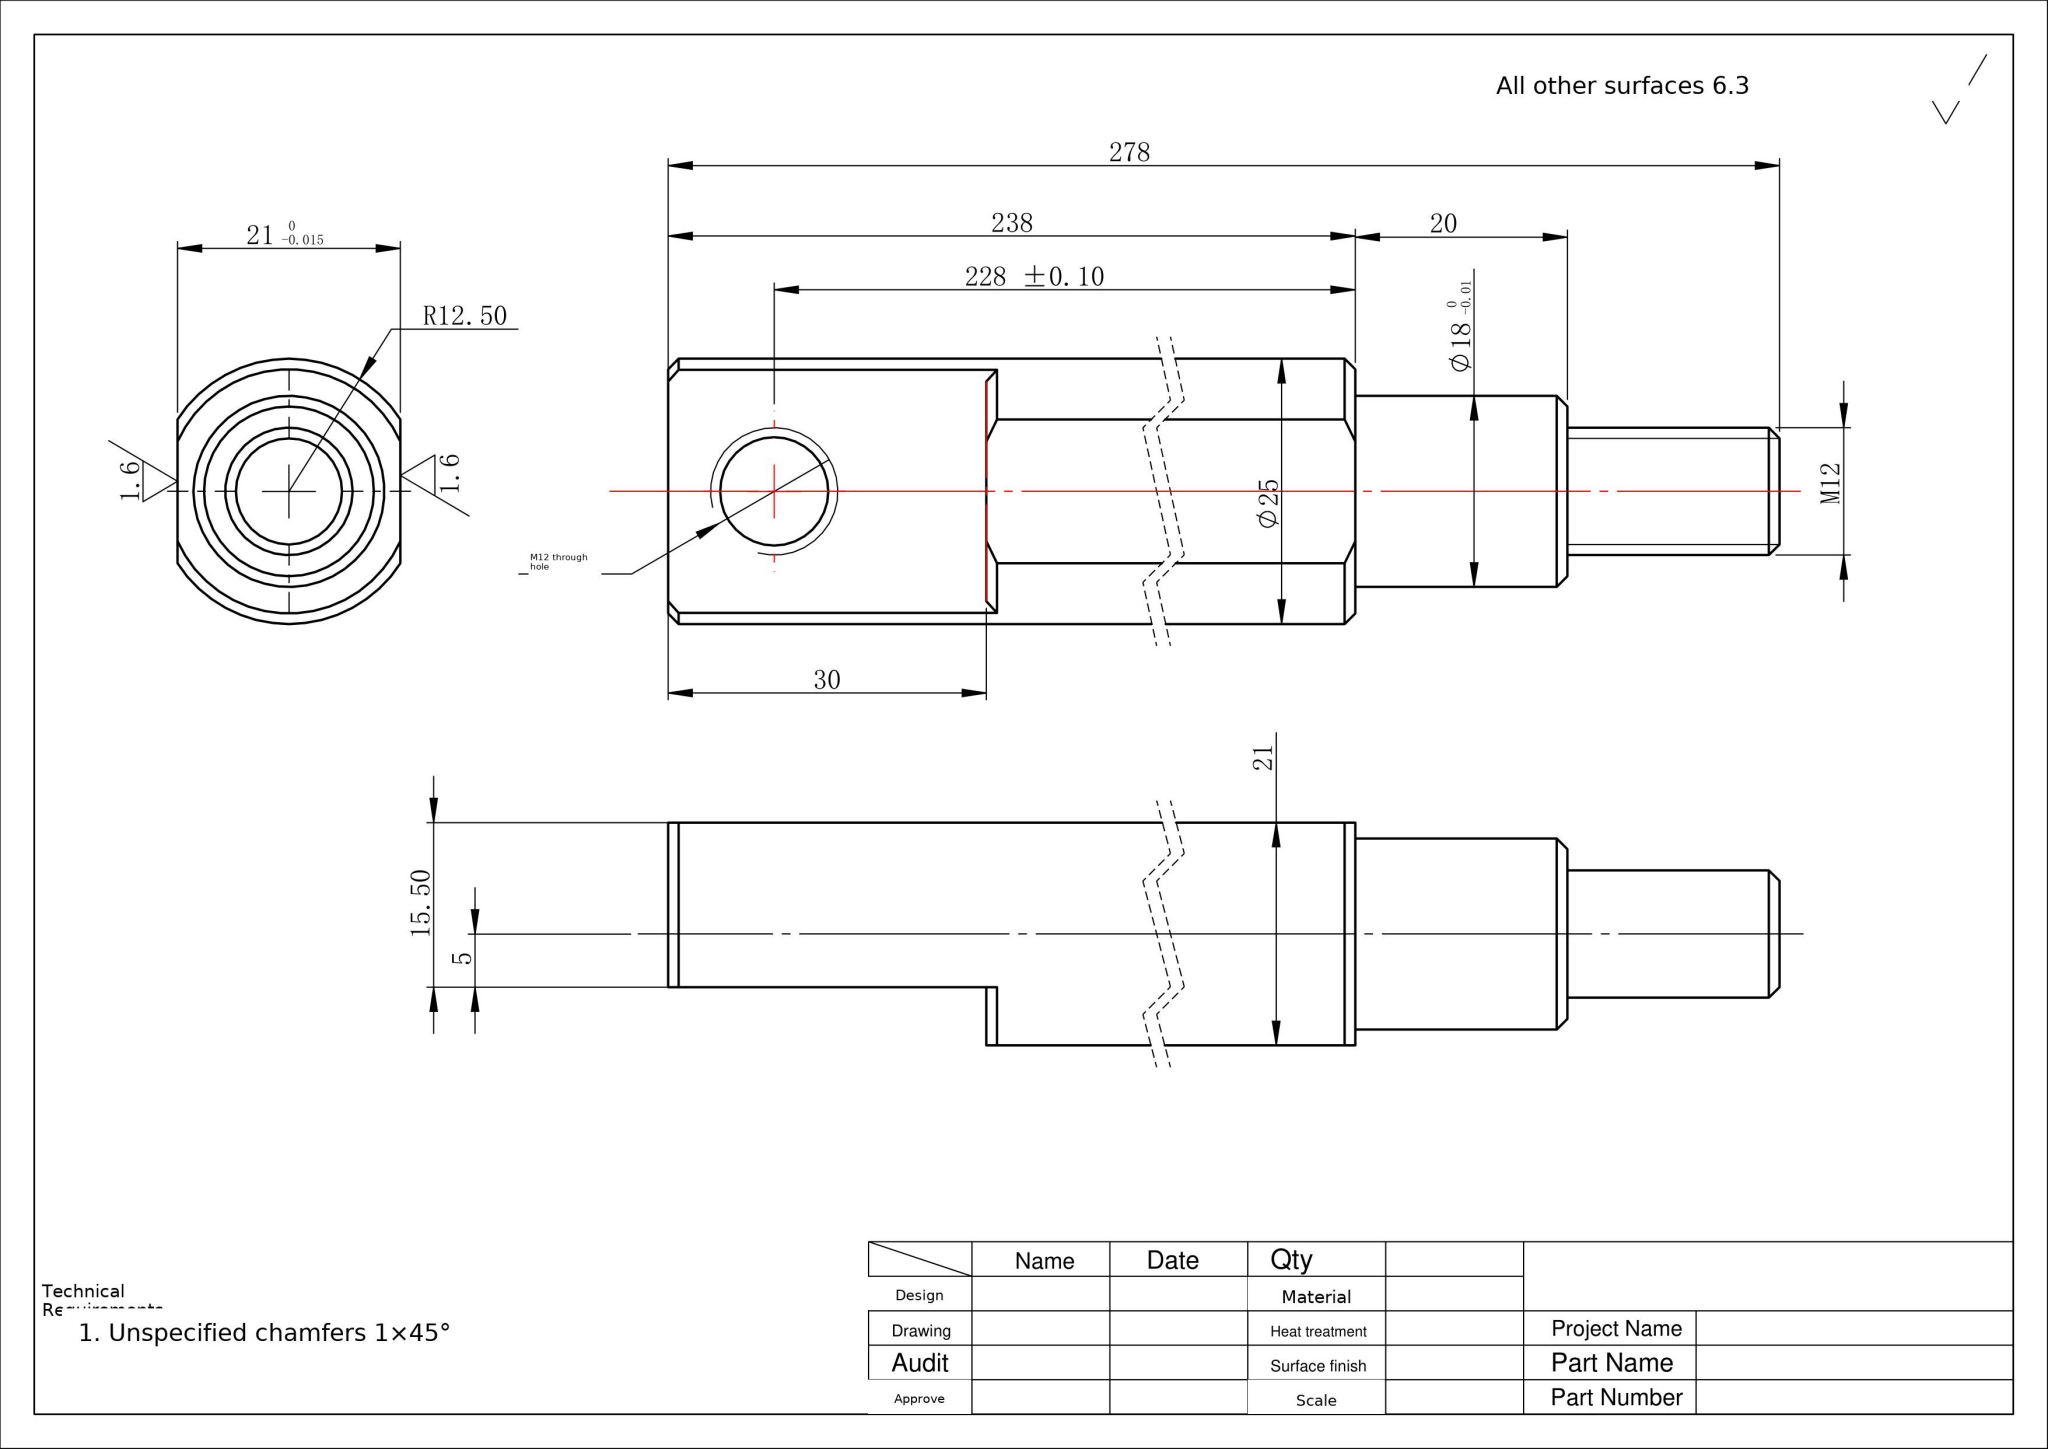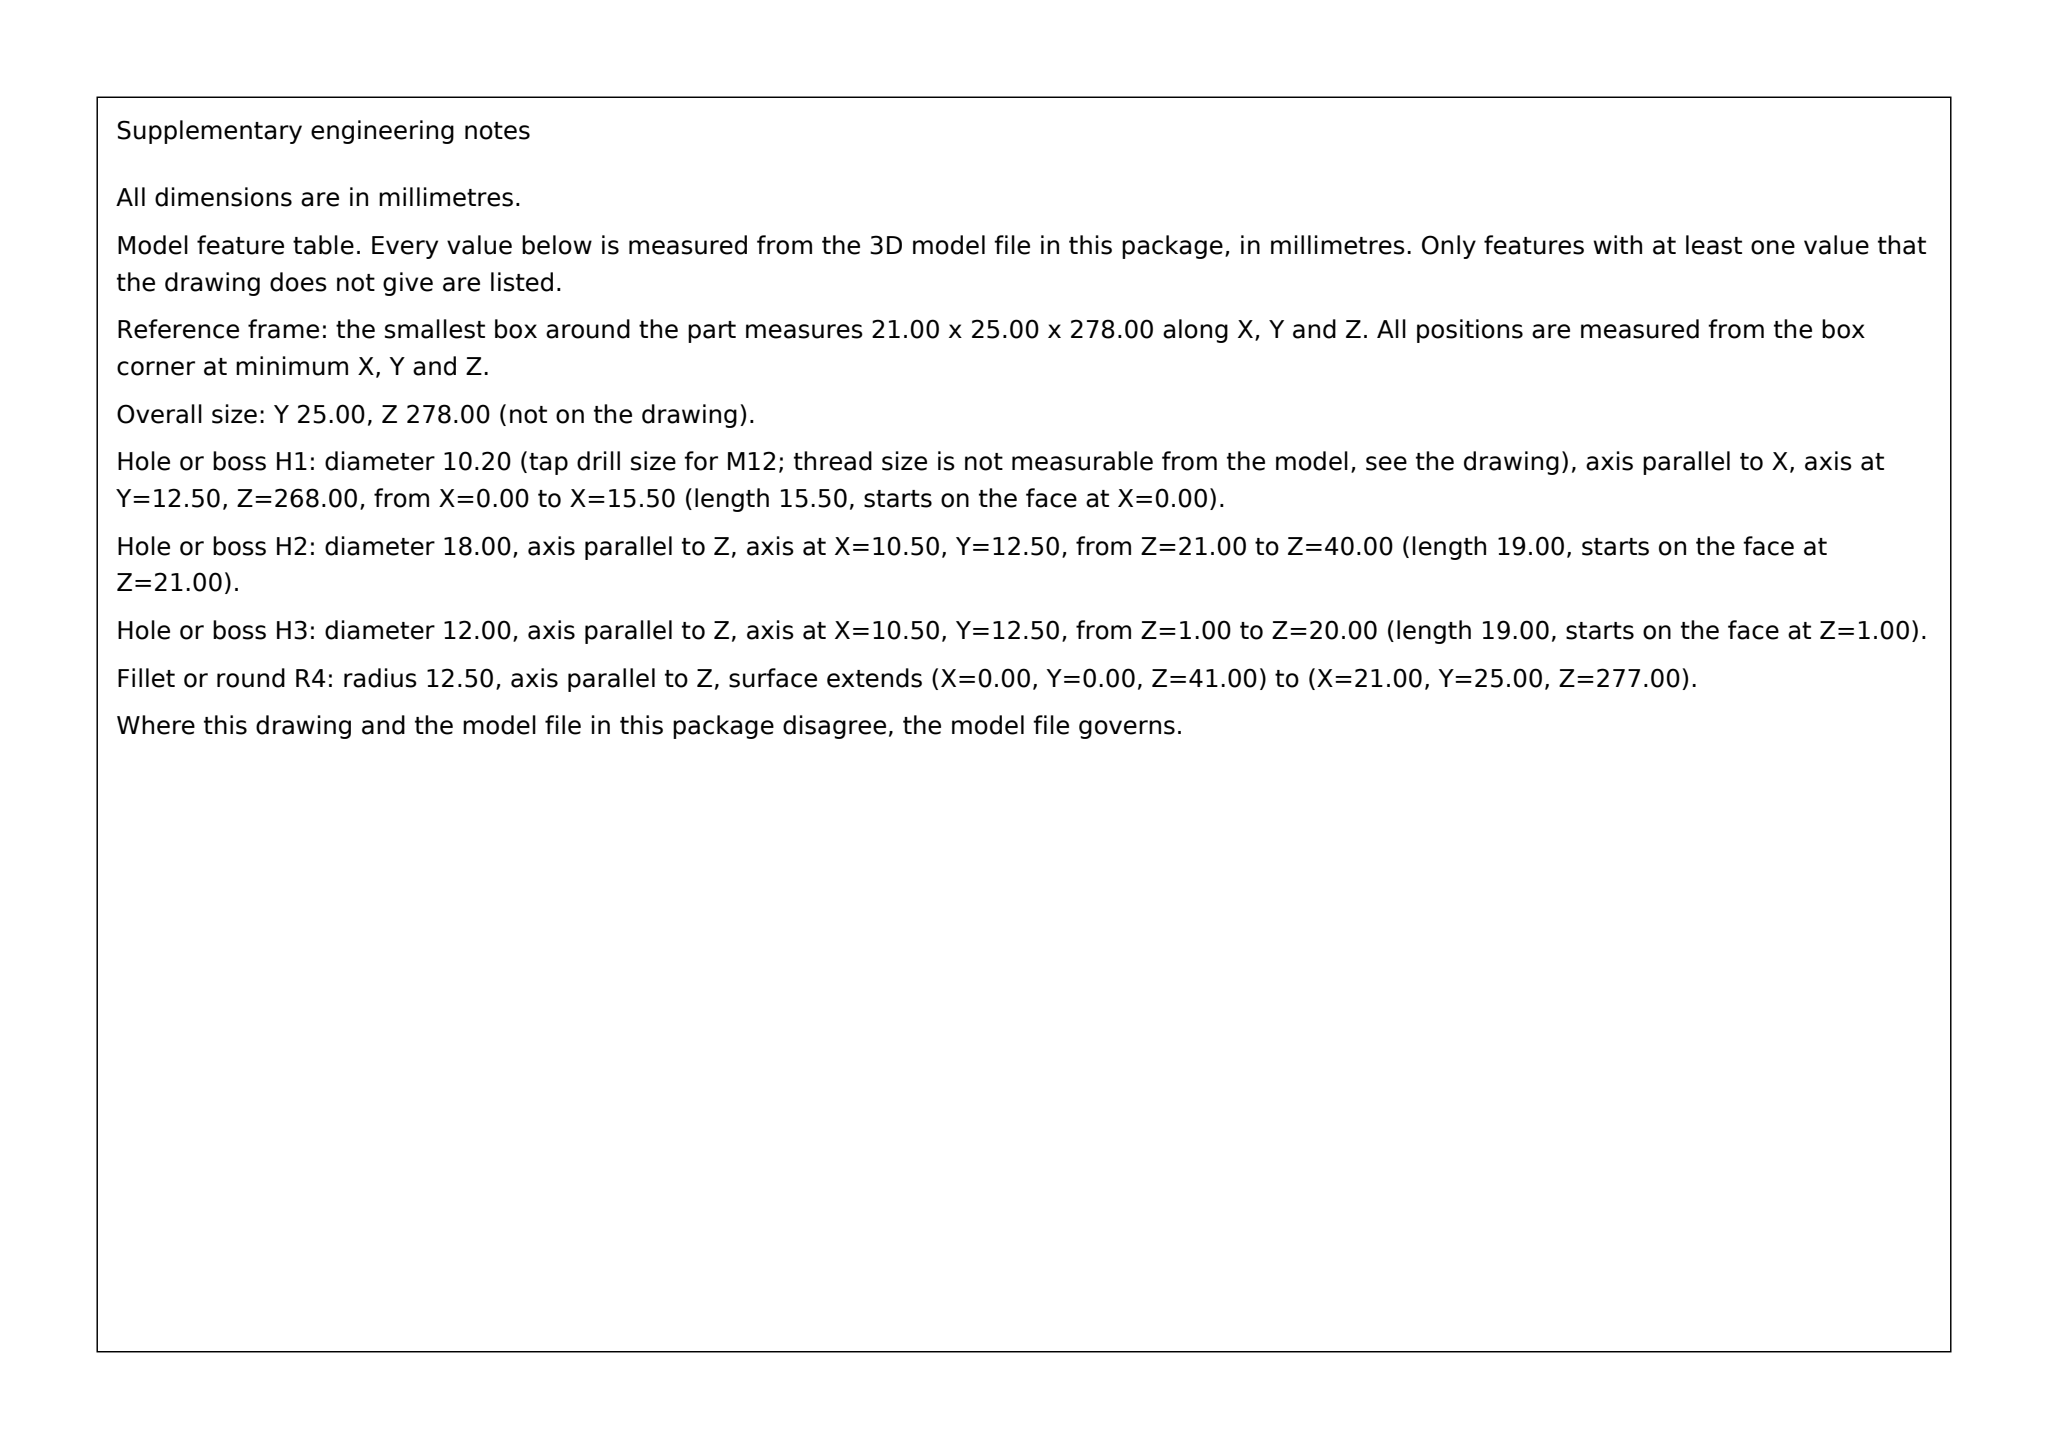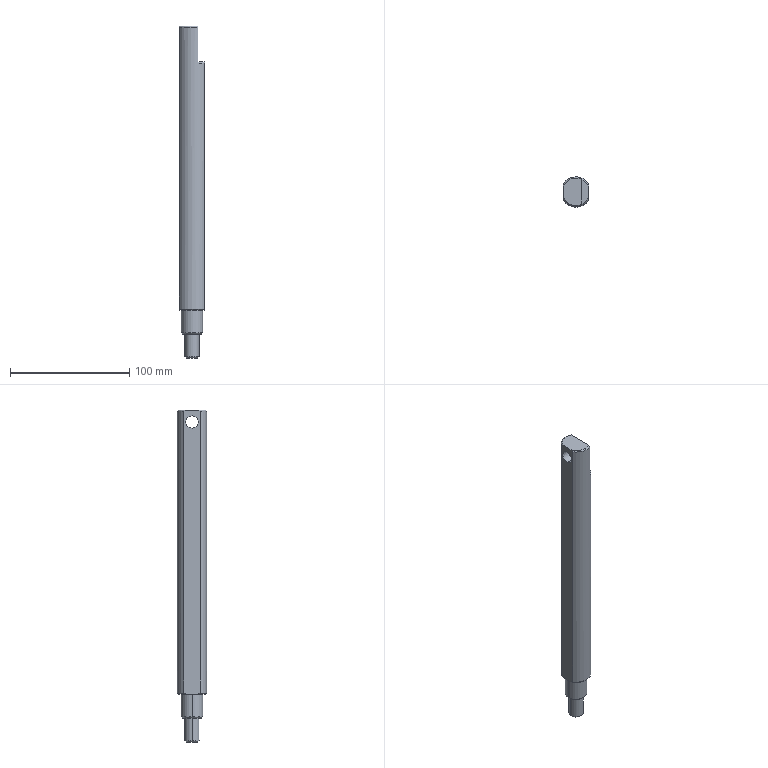Part | SolidWorks | 1 solid | 26 faces | box 21 x 25 x 278 mm | volume 110896 mm3 | cone 10 | cylinder 8 | plane 8 | commonest cylinder face diameters 12 x2 10.2 x2 18 x2 25 x2
build123d program:
from build123d import *

# Parameters (mm, degrees)
SKETCH1_R          = 9
EXTRUDE1_DEPTH     = 20
SKETCH2_R          = 12.5
EXTRUDE2_DEPTH     = 238
SKETCH6_W          = 409.623
SKETCH6_H          = 160.738
CUT_EXTRUDE2_DEPTH = 2
SKETCH7_W          = 385.784
SKETCH7_H          = 115.789
CUT_EXTRUDE3_DEPTH = 2
SKETCH8_W          = 72.586
SKETCH8_H          = 57.889
CUT_EXTRUDE4_DEPTH = 5.5
M12_TAPPED_HOLE2_D = 10.2
SKETCH11_R         = 6
EXTRUDE4_DEPTH     = 20
CHAMFER1_SIZE      = 1


with BuildPart() as part:
    # Sketch1 → Extrude1 (new body)
    with BuildSketch(Plane.XY):
        Circle(SKETCH1_R)
    extrude(amount=EXTRUDE1_DEPTH)

    # Sketch2 → Extrude2 (add)
    with BuildSketch(Plane.XY.offset(20)):
        Circle(SKETCH2_R)
    extrude(amount=EXTRUDE2_DEPTH)

    # Sketch6 → Cut-Extrude2 (cut)
    with BuildSketch(Plane(origin=(12.5, 0, 0), x_dir=(0, 0, -1), z_dir=(1, 0, 0))):
        with Locations((-133.648, -11.686)):
            Rectangle(SKETCH6_W, SKETCH6_H)
    extrude(amount=-CUT_EXTRUDE2_DEPTH, mode=Mode.SUBTRACT)

    # Sketch7 → Cut-Extrude3 (cut)
    with BuildSketch(Plane(origin=(-12.5, 0, 0), x_dir=(0, 0, -1), z_dir=(1, 0, 0))):
        with Locations((-137.977, 12.933)):
            Rectangle(SKETCH7_W, SKETCH7_H)
    extrude(amount=CUT_EXTRUDE3_DEPTH, mode=Mode.SUBTRACT)

    # Sketch8 → Cut-Extrude4 (cut)
    with BuildSketch(Plane(origin=(10.5, 0, 0), x_dir=(0, 0, -1), z_dir=(1, 0, 0))):
        with Locations((-264.293, -0.1573)):
            Rectangle(SKETCH8_W, SKETCH8_H)
    extrude(amount=-CUT_EXTRUDE4_DEPTH, mode=Mode.SUBTRACT)

    # M12 Tapped Hole2 (through all)
    with Locations(Plane(origin=(5, 0, 248), x_dir=(0, 0, 1), z_dir=(1, 0, 0))):
        with Locations((0, 0)):
            Hole(M12_TAPPED_HOLE2_D / 2)

    # Sketch11 → Extrude4 (add)
    with BuildSketch(Plane(origin=(0, 0, 0), x_dir=(-1, 0, 0), z_dir=(0, 0, -1))):
        with Locations(Location((0, 0, 0), (0, 0, 180))):
            Circle(SKETCH11_R)
    extrude(amount=EXTRUDE4_DEPTH)

    # Chamfer1
    chamfer1_edges = [part.edges().sort_by_distance(p)[0] for p in [
        (0, 12.5, 20),
        (-9, 0, 0),
        (-3.609, -11.968, 258),
        (0, -12.5, 20),
        (-3.609, 11.968, 258),
        (8.095, 9.525, 228),
        (8.095, -9.525, 228),
        (-6, 0, -20),
    ]]
    chamfer(chamfer1_edges, length=CHAMFER1_SIZE)


solid = part.part
STEP:
#1=CARTESIAN_POINT('',(-8.,0.,0.));
#2=VERTEX_POINT('',#1);
#3=CARTESIAN_POINT('',(8.,0.,0.));
#4=VERTEX_POINT('',#3);
#5=CARTESIAN_POINT('',(0.,0.,0.));
#6=DIRECTION('',(0.,0.,-1.));
#7=DIRECTION('',(1.,0.,0.));
#8=AXIS2_PLACEMENT_3D('',#5,#6,#7);
#9=CIRCLE('',#8,8.);
#10=EDGE_CURVE('',#2,#4,#9,.T.);
#11=ORIENTED_EDGE('',*,*,#10,.F.);
#12=CARTESIAN_POINT('',(-9.,0.,1.));
#13=VERTEX_POINT('',#12);
#14=CARTESIAN_POINT('',(-9.,0.,1.));
#15=DIRECTION('',(-0.7071,0.,0.7071));
#16=VECTOR('',#15,1000.);
#17=LINE('',#14,#16);
#18=EDGE_CURVE('',#2,#13,#17,.T.);
#19=ORIENTED_EDGE('',*,*,#18,.T.);
#20=CARTESIAN_POINT('',(9.,0.,1.));
#21=VERTEX_POINT('',#20);
#22=CARTESIAN_POINT('',(0.,0.,1.));
#23=DIRECTION('',(0.,0.,1.));
#24=DIRECTION('',(1.,0.,0.));
#25=AXIS2_PLACEMENT_3D('',#22,#23,#24);
#26=CIRCLE('',#25,9.);
#27=EDGE_CURVE('',#21,#13,#26,.T.);
#28=ORIENTED_EDGE('',*,*,#27,.F.);
#29=CARTESIAN_POINT('',(9.,0.,1.));
#30=DIRECTION('',(0.7071,0.,0.7071));
#31=VECTOR('',#30,1000.);
#32=LINE('',#29,#31);
#33=EDGE_CURVE('',#4,#21,#32,.T.);
#34=ORIENTED_EDGE('',*,*,#33,.F.);
#35=EDGE_LOOP('',(#11,#19,#28,#34));
#36=FACE_OUTER_BOUND('',#35,.T.);
#37=CARTESIAN_POINT('',(0.,0.,1.));
#38=DIRECTION('',(0.,0.,1.));
#39=DIRECTION('',(1.,0.,0.));
#40=AXIS2_PLACEMENT_3D('',#37,#38,#39);
#41=CONICAL_SURFACE('',#40,9.,0.7854);
#42=ADVANCED_FACE('',(#36),#41,.T.);
#43=CARTESIAN_POINT('',(-5.,0.,-20.));
#44=VERTEX_POINT('',#43);
#45=CARTESIAN_POINT('',(5.,0.,-20.));
#46=VERTEX_POINT('',#45);
#47=CARTESIAN_POINT('',(0.,0.,-20.));
#48=DIRECTION('',(0.,0.,-1.));
#49=DIRECTION('',(-1.,0.,0.));
#50=AXIS2_PLACEMENT_3D('',#47,#48,#49);
#51=CIRCLE('',#50,5.);
#52=EDGE_CURVE('',#44,#46,#51,.T.);
#53=ORIENTED_EDGE('',*,*,#52,.F.);
#54=CARTESIAN_POINT('',(-6.,0.,-19.));
#55=VERTEX_POINT('',#54);
#56=CARTESIAN_POINT('',(-5.,0.,-20.));
#57=DIRECTION('',(-0.7071,0.,0.7071));
#58=VECTOR('',#57,1000.);
#59=LINE('',#56,#58);
#60=EDGE_CURVE('',#44,#55,#59,.T.);
#61=ORIENTED_EDGE('',*,*,#60,.T.);
#62=CARTESIAN_POINT('',(6.,0.,-19.));
#63=VERTEX_POINT('',#62);
#64=CARTESIAN_POINT('',(0.,0.,-19.));
#65=DIRECTION('',(0.,0.,1.));
#66=DIRECTION('',(-1.,0.,0.));
#67=AXIS2_PLACEMENT_3D('',#64,#65,#66);
#68=CIRCLE('',#67,6.);
#69=EDGE_CURVE('',#63,#55,#68,.T.);
#70=ORIENTED_EDGE('',*,*,#69,.F.);
#71=CARTESIAN_POINT('',(5.,0.,-20.));
#72=DIRECTION('',(0.7071,0.,0.7071));
#73=VECTOR('',#72,1000.);
#74=LINE('',#71,#73);
#75=EDGE_CURVE('',#46,#63,#74,.T.);
#76=ORIENTED_EDGE('',*,*,#75,.F.);
#77=EDGE_LOOP('',(#53,#61,#70,#76));
#78=FACE_OUTER_BOUND('',#77,.T.);
#79=CARTESIAN_POINT('',(0.,0.,-20.));
#80=DIRECTION('',(0.,0.,1.));
#81=DIRECTION('',(1.,0.,0.));
#82=AXIS2_PLACEMENT_3D('',#79,#80,#81);
#83=CONICAL_SURFACE('',#82,5.,0.7854);
#84=ADVANCED_FACE('',(#78),#83,.T.);
#85=ORIENTED_EDGE('',*,*,#69,.T.);
#86=CARTESIAN_POINT('',(-6.,0.,0.));
#87=VERTEX_POINT('',#86);
#88=CARTESIAN_POINT('',(-6.,0.,-20.));
#89=DIRECTION('',(0.,0.,1.));
#90=VECTOR('',#89,1000.);
#91=LINE('',#88,#90);
#92=EDGE_CURVE('',#55,#87,#91,.T.);
#93=ORIENTED_EDGE('',*,*,#92,.T.);
#94=CARTESIAN_POINT('',(6.,0.,0.));
#95=VERTEX_POINT('',#94);
#96=CARTESIAN_POINT('',(0.,0.,0.));
#97=DIRECTION('',(0.,0.,-1.));
#98=DIRECTION('',(1.,0.,0.));
#99=AXIS2_PLACEMENT_3D('',#96,#97,#98);
#100=CIRCLE('',#99,6.);
#101=EDGE_CURVE('',#87,#95,#100,.T.);
#102=ORIENTED_EDGE('',*,*,#101,.T.);
#103=CARTESIAN_POINT('',(6.,0.,-20.));
#104=DIRECTION('',(0.,0.,1.));
#105=VECTOR('',#104,1000.);
#106=LINE('',#103,#105);
#107=EDGE_CURVE('',#63,#95,#106,.T.);
#108=ORIENTED_EDGE('',*,*,#107,.F.);
#109=EDGE_LOOP('',(#85,#93,#102,#108));
#110=FACE_OUTER_BOUND('',#109,.T.);
#111=CARTESIAN_POINT('',(0.,0.,-20.));
#112=DIRECTION('',(0.,0.,1.));
#113=DIRECTION('',(1.,0.,0.));
#114=AXIS2_PLACEMENT_3D('',#111,#112,#113);
#115=CYLINDRICAL_SURFACE('',#114,6.);
#116=ADVANCED_FACE('',(#110),#115,.T.);
#117=CARTESIAN_POINT('',(-10.5,0.,253.1));
#118=VERTEX_POINT('',#117);
#119=CARTESIAN_POINT('',(-10.5,0.,242.9));
#120=VERTEX_POINT('',#119);
#121=CARTESIAN_POINT('',(-10.5,0.,248.));
#122=DIRECTION('',(1.,0.,0.));
#123=DIRECTION('',(0.,0.,-1.));
#124=AXIS2_PLACEMENT_3D('',#121,#122,#123);
#125=CIRCLE('',#124,5.1);
#126=EDGE_CURVE('',#118,#120,#125,.T.);
#127=ORIENTED_EDGE('',*,*,#126,.F.);
#128=CARTESIAN_POINT('',(5.,0.,253.1));
#129=VERTEX_POINT('',#128);
#130=CARTESIAN_POINT('',(5.,0.,253.1));
#131=DIRECTION('',(1.,0.,0.));
#132=VECTOR('',#131,1000.);
#133=LINE('',#130,#132);
#134=EDGE_CURVE('',#118,#129,#133,.T.);
#135=ORIENTED_EDGE('',*,*,#134,.T.);
#136=CARTESIAN_POINT('',(5.,0.,242.9));
#137=VERTEX_POINT('',#136);
#138=CARTESIAN_POINT('',(5.,0.,248.));
#139=DIRECTION('',(1.,0.,0.));
#140=DIRECTION('',(0.,0.,-1.));
#141=AXIS2_PLACEMENT_3D('',#138,#139,#140);
#142=CIRCLE('',#141,5.1);
#143=EDGE_CURVE('',#129,#137,#142,.T.);
#144=ORIENTED_EDGE('',*,*,#143,.T.);
#145=CARTESIAN_POINT('',(5.,0.,242.9));
#146=DIRECTION('',(1.,0.,0.));
#147=VECTOR('',#146,1000.);
#148=LINE('',#145,#147);
#149=EDGE_CURVE('',#120,#137,#148,.T.);
#150=ORIENTED_EDGE('',*,*,#149,.F.);
#151=EDGE_LOOP('',(#127,#135,#144,#150));
#152=FACE_OUTER_BOUND('',#151,.T.);
#153=CARTESIAN_POINT('',(5.,0.,248.));
#154=DIRECTION('',(1.,0.,0.));
#155=DIRECTION('',(0.,0.,-1.));
#156=AXIS2_PLACEMENT_3D('',#153,#154,#155);
#157=CYLINDRICAL_SURFACE('',#156,5.1);
#158=ADVANCED_FACE('',(#152),#157,.F.);
#159=CARTESIAN_POINT('',(9.,0.,20.));
#160=VERTEX_POINT('',#159);
#161=CARTESIAN_POINT('',(-9.,0.,20.));
#162=VERTEX_POINT('',#161);
#163=CARTESIAN_POINT('',(0.,0.,20.));
#164=DIRECTION('',(0.,0.,1.));
#165=DIRECTION('',(1.,0.,0.));
#166=AXIS2_PLACEMENT_3D('',#163,#164,#165);
#167=CIRCLE('',#166,9.);
#168=EDGE_CURVE('',#160,#162,#167,.T.);
#169=ORIENTED_EDGE('',*,*,#168,.F.);
#170=CARTESIAN_POINT('',(9.,0.,20.));
#171=DIRECTION('',(0.,0.,-1.));
#172=VECTOR('',#171,1000.);
#173=LINE('',#170,#172);
#174=EDGE_CURVE('',#160,#21,#173,.T.);
#175=ORIENTED_EDGE('',*,*,#174,.T.);
#176=ORIENTED_EDGE('',*,*,#27,.T.);
#177=CARTESIAN_POINT('',(-9.,0.,20.));
#178=DIRECTION('',(0.,0.,-1.));
#179=VECTOR('',#178,1000.);
#180=LINE('',#177,#179);
#181=EDGE_CURVE('',#162,#13,#180,.T.);
#182=ORIENTED_EDGE('',*,*,#181,.F.);
#183=EDGE_LOOP('',(#169,#175,#176,#182));
#184=FACE_OUTER_BOUND('',#183,.T.);
#185=CARTESIAN_POINT('',(0.,0.,20.));
#186=DIRECTION('',(0.,0.,-1.));
#187=DIRECTION('',(-1.,0.,0.));
#188=AXIS2_PLACEMENT_3D('',#185,#186,#187);
#189=CYLINDRICAL_SURFACE('',#188,9.);
#190=ADVANCED_FACE('',(#184),#189,.T.);
#191=CARTESIAN_POINT('',(0.,0.,0.));
#192=DIRECTION('',(0.,0.,-1.));
#193=DIRECTION('',(1.,0.,0.));
#194=AXIS2_PLACEMENT_3D('',#191,#192,#193);
#195=CIRCLE('',#194,8.);
#196=EDGE_CURVE('',#4,#2,#195,.T.);
#197=ORIENTED_EDGE('',*,*,#196,.T.);
#198=ORIENTED_EDGE('',*,*,#10,.T.);
#199=EDGE_LOOP('',(#197,#198));
#200=FACE_OUTER_BOUND('',#199,.T.);
#201=CARTESIAN_POINT('',(0.,0.,0.));
#202=DIRECTION('',(0.,0.,-1.));
#203=DIRECTION('',(1.,0.,0.));
#204=AXIS2_PLACEMENT_3D('',#201,#202,#203);
#205=CIRCLE('',#204,6.);
#206=EDGE_CURVE('',#95,#87,#205,.T.);
#207=ORIENTED_EDGE('',*,*,#206,.F.);
#208=ORIENTED_EDGE('',*,*,#101,.F.);
#209=EDGE_LOOP('',(#207,#208));
#210=FACE_BOUND('',#209,.T.);
#211=CARTESIAN_POINT('',(0.,0.,0.));
#212=DIRECTION('',(0.,0.,1.));
#213=DIRECTION('',(1.,0.,0.));
#214=AXIS2_PLACEMENT_3D('',#211,#212,#213);
#215=PLANE('',#214);
#216=ADVANCED_FACE('',(#200,#210),#215,.F.);
#217=CARTESIAN_POINT('',(5.,11.456,257.));
#218=VERTEX_POINT('',#217);
#219=CARTESIAN_POINT('',(5.,11.456,227.));
#220=VERTEX_POINT('',#219);
#221=CARTESIAN_POINT('',(5.,11.456,258.));
#222=DIRECTION('',(0.,0.,-1.));
#223=VECTOR('',#222,1000.);
#224=LINE('',#221,#223);
#225=EDGE_CURVE('',#218,#220,#224,.T.);
#226=ORIENTED_EDGE('',*,*,#225,.T.);
#227=CARTESIAN_POINT('',(10.5,6.782,227.));
#228=VERTEX_POINT('',#227);
#229=CARTESIAN_POINT('',(0.,0.,227.));
#230=DIRECTION('',(0.,0.,-1.));
#231=DIRECTION('',(-1.,0.,0.));
#232=AXIS2_PLACEMENT_3D('',#229,#230,#231);
#233=CIRCLE('',#232,12.5);
#234=EDGE_CURVE('',#220,#228,#233,.T.);
#235=ORIENTED_EDGE('',*,*,#234,.T.);
#236=CARTESIAN_POINT('',(10.5,6.782,21.));
#237=VERTEX_POINT('',#236);
#238=CARTESIAN_POINT('',(10.5,6.782,258.));
#239=DIRECTION('',(0.,0.,-1.));
#240=VECTOR('',#239,1000.);
#241=LINE('',#238,#240);
#242=EDGE_CURVE('',#228,#237,#241,.T.);
#243=ORIENTED_EDGE('',*,*,#242,.T.);
#244=CARTESIAN_POINT('',(-10.5,6.782,21.));
#245=VERTEX_POINT('',#244);
#246=CARTESIAN_POINT('',(0.,0.,21.));
#247=DIRECTION('',(0.,0.,1.));
#248=DIRECTION('',(1.,0.,0.));
#249=AXIS2_PLACEMENT_3D('',#246,#247,#248);
#250=CIRCLE('',#249,12.5);
#251=EDGE_CURVE('',#237,#245,#250,.T.);
#252=ORIENTED_EDGE('',*,*,#251,.T.);
#253=CARTESIAN_POINT('',(-10.5,6.782,257.));
#254=VERTEX_POINT('',#253);
#255=CARTESIAN_POINT('',(-10.5,6.782,258.));
#256=DIRECTION('',(0.,0.,1.));
#257=VECTOR('',#256,1000.);
#258=LINE('',#255,#257);
#259=EDGE_CURVE('',#245,#254,#258,.T.);
#260=ORIENTED_EDGE('',*,*,#259,.T.);
#261=CARTESIAN_POINT('',(0.,0.,257.));
#262=DIRECTION('',(0.,0.,-1.));
#263=DIRECTION('',(1.,0.,0.));
#264=AXIS2_PLACEMENT_3D('',#261,#262,#263);
#265=CIRCLE('',#264,12.5);
#266=EDGE_CURVE('',#254,#218,#265,.T.);
#267=ORIENTED_EDGE('',*,*,#266,.T.);
#268=EDGE_LOOP('',(#226,#235,#243,#252,#260,#267));
#269=FACE_OUTER_BOUND('',#268,.T.);
#270=CARTESIAN_POINT('',(0.,0.,258.));
#271=DIRECTION('',(0.,0.,-1.));
#272=DIRECTION('',(-1.,0.,0.));
#273=AXIS2_PLACEMENT_3D('',#270,#271,#272);
#274=CYLINDRICAL_SURFACE('',#273,12.5);
#275=ADVANCED_FACE('',(#269),#274,.T.);
#276=ORIENTED_EDGE('',*,*,#174,.F.);
#277=CARTESIAN_POINT('',(0.,0.,20.));
#278=DIRECTION('',(0.,0.,1.));
#279=DIRECTION('',(1.,0.,0.));
#280=AXIS2_PLACEMENT_3D('',#277,#278,#279);
#281=CIRCLE('',#280,9.);
#282=EDGE_CURVE('',#162,#160,#281,.T.);
#283=ORIENTED_EDGE('',*,*,#282,.F.);
#284=ORIENTED_EDGE('',*,*,#181,.T.);
#285=CARTESIAN_POINT('',(0.,0.,1.));
#286=DIRECTION('',(0.,0.,1.));
#287=DIRECTION('',(1.,0.,0.));
#288=AXIS2_PLACEMENT_3D('',#285,#286,#287);
#289=CIRCLE('',#288,9.);
#290=EDGE_CURVE('',#13,#21,#289,.T.);
#291=ORIENTED_EDGE('',*,*,#290,.T.);
#292=EDGE_LOOP('',(#276,#283,#284,#291));
#293=FACE_OUTER_BOUND('',#292,.T.);
#294=CARTESIAN_POINT('',(0.,0.,20.));
#295=DIRECTION('',(0.,0.,-1.));
#296=DIRECTION('',(-1.,0.,0.));
#297=AXIS2_PLACEMENT_3D('',#294,#295,#296);
#298=CYLINDRICAL_SURFACE('',#297,9.);
#299=ADVANCED_FACE('',(#293),#298,.T.);
#300=CARTESIAN_POINT('',(-10.5,-4.69,20.));
#301=VERTEX_POINT('',#300);
#302=CARTESIAN_POINT('',(-10.5,4.69,20.));
#303=VERTEX_POINT('',#302);
#304=CARTESIAN_POINT('',(-10.5,0.,20.));
#305=DIRECTION('',(0.,1.,0.));
#306=VECTOR('',#305,1000.);
#307=LINE('',#304,#306);
#308=EDGE_CURVE('',#301,#303,#307,.T.);
#309=ORIENTED_EDGE('',*,*,#308,.T.);
#310=CARTESIAN_POINT('',(10.5,4.69,20.));
#311=VERTEX_POINT('',#310);
#312=CARTESIAN_POINT('',(0.,0.,20.));
#313=DIRECTION('',(0.,0.,-1.));
#314=DIRECTION('',(1.,0.,0.));
#315=AXIS2_PLACEMENT_3D('',#312,#313,#314);
#316=CIRCLE('',#315,11.5);
#317=EDGE_CURVE('',#303,#311,#316,.T.);
#318=ORIENTED_EDGE('',*,*,#317,.T.);
#319=CARTESIAN_POINT('',(10.5,-4.69,20.));
#320=VERTEX_POINT('',#319);
#321=CARTESIAN_POINT('',(10.5,0.,20.));
#322=DIRECTION('',(0.,-1.,0.));
#323=VECTOR('',#322,1000.);
#324=LINE('',#321,#323);
#325=EDGE_CURVE('',#311,#320,#324,.T.);
#326=ORIENTED_EDGE('',*,*,#325,.T.);
#327=CARTESIAN_POINT('',(0.,0.,20.));
#328=DIRECTION('',(0.,0.,-1.));
#329=DIRECTION('',(1.,0.,0.));
#330=AXIS2_PLACEMENT_3D('',#327,#328,#329);
#331=CIRCLE('',#330,11.5);
#332=EDGE_CURVE('',#320,#301,#331,.T.);
#333=ORIENTED_EDGE('',*,*,#332,.T.);
#334=EDGE_LOOP('',(#309,#318,#326,#333));
#335=FACE_OUTER_BOUND('',#334,.T.);
#336=ORIENTED_EDGE('',*,*,#282,.T.);
#337=ORIENTED_EDGE('',*,*,#168,.T.);
#338=EDGE_LOOP('',(#336,#337));
#339=FACE_BOUND('',#338,.T.);
#340=CARTESIAN_POINT('',(0.,0.,20.));
#341=DIRECTION('',(0.,0.,1.));
#342=DIRECTION('',(1.,0.,0.));
#343=AXIS2_PLACEMENT_3D('',#340,#341,#342);
#344=PLANE('',#343);
#345=ADVANCED_FACE('',(#335,#339),#344,.F.);
#346=CARTESIAN_POINT('',(10.5,-6.782,21.));
#347=VERTEX_POINT('',#346);
#348=CARTESIAN_POINT('',(10.5,-6.782,227.));
#349=VERTEX_POINT('',#348);
#350=CARTESIAN_POINT('',(10.5,-6.782,258.));
#351=DIRECTION('',(0.,0.,1.));
#352=VECTOR('',#351,1000.);
#353=LINE('',#350,#352);
#354=EDGE_CURVE('',#347,#349,#353,.T.);
#355=ORIENTED_EDGE('',*,*,#354,.T.);
#356=CARTESIAN_POINT('',(5.,-11.456,227.));
#357=VERTEX_POINT('',#356);
#358=CARTESIAN_POINT('',(0.,0.,227.));
#359=DIRECTION('',(0.,0.,-1.));
#360=DIRECTION('',(-1.,0.,0.));
#361=AXIS2_PLACEMENT_3D('',#358,#359,#360);
#362=CIRCLE('',#361,12.5);
#363=EDGE_CURVE('',#349,#357,#362,.T.);
#364=ORIENTED_EDGE('',*,*,#363,.T.);
#365=CARTESIAN_POINT('',(5.,-11.456,257.));
#366=VERTEX_POINT('',#365);
#367=CARTESIAN_POINT('',(5.,-11.456,258.));
#368=DIRECTION('',(0.,0.,1.));
#369=VECTOR('',#368,1000.);
#370=LINE('',#367,#369);
#371=EDGE_CURVE('',#357,#366,#370,.T.);
#372=ORIENTED_EDGE('',*,*,#371,.T.);
#373=CARTESIAN_POINT('',(-10.5,-6.782,257.));
#374=VERTEX_POINT('',#373);
#375=CARTESIAN_POINT('',(0.,0.,257.));
#376=DIRECTION('',(0.,0.,-1.));
#377=DIRECTION('',(1.,0.,0.));
#378=AXIS2_PLACEMENT_3D('',#375,#376,#377);
#379=CIRCLE('',#378,12.5);
#380=EDGE_CURVE('',#366,#374,#379,.T.);
#381=ORIENTED_EDGE('',*,*,#380,.T.);
#382=CARTESIAN_POINT('',(-10.5,-6.782,21.));
#383=VERTEX_POINT('',#382);
#384=CARTESIAN_POINT('',(-10.5,-6.782,258.));
#385=DIRECTION('',(0.,0.,-1.));
#386=VECTOR('',#385,1000.);
#387=LINE('',#384,#386);
#388=EDGE_CURVE('',#374,#383,#387,.T.);
#389=ORIENTED_EDGE('',*,*,#388,.T.);
#390=CARTESIAN_POINT('',(0.,0.,21.));
#391=DIRECTION('',(0.,0.,1.));
#392=DIRECTION('',(1.,0.,0.));
#393=AXIS2_PLACEMENT_3D('',#390,#391,#392);
#394=CIRCLE('',#393,12.5);
#395=EDGE_CURVE('',#383,#347,#394,.T.);
#396=ORIENTED_EDGE('',*,*,#395,.T.);
#397=EDGE_LOOP('',(#355,#364,#372,#381,#389,#396));
#398=FACE_OUTER_BOUND('',#397,.T.);
#399=CARTESIAN_POINT('',(0.,0.,258.));
#400=DIRECTION('',(0.,0.,-1.));
#401=DIRECTION('',(-1.,0.,0.));
#402=AXIS2_PLACEMENT_3D('',#399,#400,#401);
#403=CYLINDRICAL_SURFACE('',#402,12.5);
#404=ADVANCED_FACE('',(#398),#403,.T.);
#405=CARTESIAN_POINT('',(-10.5,-4.69,258.));
#406=VERTEX_POINT('',#405);
#407=CARTESIAN_POINT('',(-10.5,4.69,258.));
#408=VERTEX_POINT('',#407);
#409=CARTESIAN_POINT('',(-10.5,0.,258.));
#410=DIRECTION('',(0.,1.,0.));
#411=VECTOR('',#410,1000.);
#412=LINE('',#409,#411);
#413=EDGE_CURVE('',#406,#408,#412,.T.);
#414=ORIENTED_EDGE('',*,*,#413,.F.);
#415=CARTESIAN_POINT('',(5.,-10.356,258.));
#416=VERTEX_POINT('',#415);
#417=CARTESIAN_POINT('',(0.,0.,258.));
#418=DIRECTION('',(0.,0.,1.));
#419=DIRECTION('',(1.,0.,0.));
#420=AXIS2_PLACEMENT_3D('',#417,#418,#419);
#421=CIRCLE('',#420,11.5);
#422=EDGE_CURVE('',#406,#416,#421,.T.);
#423=ORIENTED_EDGE('',*,*,#422,.T.);
#424=CARTESIAN_POINT('',(5.,10.356,258.));
#425=VERTEX_POINT('',#424);
#426=CARTESIAN_POINT('',(5.,0.,258.));
#427=DIRECTION('',(0.,-1.,0.));
#428=VECTOR('',#427,1000.);
#429=LINE('',#426,#428);
#430=EDGE_CURVE('',#425,#416,#429,.T.);
#431=ORIENTED_EDGE('',*,*,#430,.F.);
#432=CARTESIAN_POINT('',(0.,0.,258.));
#433=DIRECTION('',(0.,0.,1.));
#434=DIRECTION('',(1.,0.,0.));
#435=AXIS2_PLACEMENT_3D('',#432,#433,#434);
#436=CIRCLE('',#435,11.5);
#437=EDGE_CURVE('',#425,#408,#436,.T.);
#438=ORIENTED_EDGE('',*,*,#437,.T.);
#439=EDGE_LOOP('',(#414,#423,#431,#438));
#440=FACE_OUTER_BOUND('',#439,.T.);
#441=CARTESIAN_POINT('',(0.,0.,258.));
#442=DIRECTION('',(0.,0.,1.));
#443=DIRECTION('',(1.,0.,0.));
#444=AXIS2_PLACEMENT_3D('',#441,#442,#443);
#445=PLANE('',#444);
#446=ADVANCED_FACE('',(#440),#445,.T.);
#447=CARTESIAN_POINT('',(10.5,4.69,228.));
#448=VERTEX_POINT('',#447);
#449=CARTESIAN_POINT('',(10.5,-4.69,228.));
#450=VERTEX_POINT('',#449);
#451=CARTESIAN_POINT('',(10.5,68.683,228.));
#452=DIRECTION('',(0.,-1.,0.));
#453=VECTOR('',#452,1000.);
#454=LINE('',#451,#453);
#455=EDGE_CURVE('',#448,#450,#454,.T.);
#456=ORIENTED_EDGE('',*,*,#455,.T.);
#457=CARTESIAN_POINT('',(10.5,-4.69,228.));
#458=CARTESIAN_POINT('',(10.5,-5.407,227.708));
#459=CARTESIAN_POINT('',(10.5,-6.102,227.369));
#460=CARTESIAN_POINT('',(10.5,-6.782,227.));
#461=B_SPLINE_CURVE_WITH_KNOTS('',3,(#457,#458,#459,#460),.UNSPECIFIED.,.F.,.F.,(4,4),(0.,0.002319),.UNSPECIFIED.);
#462=EDGE_CURVE('',#450,#349,#461,.T.);
#463=ORIENTED_EDGE('',*,*,#462,.T.);
#464=ORIENTED_EDGE('',*,*,#354,.F.);
#465=CARTESIAN_POINT('',(10.5,-6.782,21.));
#466=CARTESIAN_POINT('',(10.5,-6.102,20.631));
#467=CARTESIAN_POINT('',(10.5,-5.407,20.292));
#468=CARTESIAN_POINT('',(10.5,-4.69,20.));
#469=B_SPLINE_CURVE_WITH_KNOTS('',3,(#465,#466,#467,#468),.UNSPECIFIED.,.F.,.F.,(4,4),(0.,0.002319),.UNSPECIFIED.);
#470=EDGE_CURVE('',#347,#320,#469,.T.);
#471=ORIENTED_EDGE('',*,*,#470,.T.);
#472=ORIENTED_EDGE('',*,*,#325,.F.);
#473=CARTESIAN_POINT('',(10.5,4.69,20.));
#474=CARTESIAN_POINT('',(10.5,5.407,20.292));
#475=CARTESIAN_POINT('',(10.5,6.102,20.631));
#476=CARTESIAN_POINT('',(10.5,6.782,21.));
#477=B_SPLINE_CURVE_WITH_KNOTS('',3,(#473,#474,#475,#476),.UNSPECIFIED.,.F.,.F.,(4,4),(0.,0.002319),.UNSPECIFIED.);
#478=EDGE_CURVE('',#311,#237,#477,.T.);
#479=ORIENTED_EDGE('',*,*,#478,.T.);
#480=ORIENTED_EDGE('',*,*,#242,.F.);
#481=CARTESIAN_POINT('',(10.5,6.782,227.));
#482=CARTESIAN_POINT('',(10.5,6.102,227.369));
#483=CARTESIAN_POINT('',(10.5,5.407,227.708));
#484=CARTESIAN_POINT('',(10.5,4.69,228.));
#485=B_SPLINE_CURVE_WITH_KNOTS('',3,(#481,#482,#483,#484),.UNSPECIFIED.,.F.,.F.,(4,4),(0.,0.002319),.UNSPECIFIED.);
#486=EDGE_CURVE('',#228,#448,#485,.T.);
#487=ORIENTED_EDGE('',*,*,#486,.T.);
#488=EDGE_LOOP('',(#456,#463,#464,#471,#472,#479,#480,#487));
#489=FACE_OUTER_BOUND('',#488,.T.);
#490=CARTESIAN_POINT('',(10.5,68.683,338.46));
#491=DIRECTION('',(-1.,0.,0.));
#492=DIRECTION('',(0.,0.,1.));
#493=AXIS2_PLACEMENT_3D('',#490,#491,#492);
#494=PLANE('',#493);
#495=ADVANCED_FACE('',(#489),#494,.F.);
#496=CARTESIAN_POINT('',(-10.5,0.,248.));
#497=DIRECTION('',(1.,0.,0.));
#498=DIRECTION('',(0.,0.,-1.));
#499=AXIS2_PLACEMENT_3D('',#496,#497,#498);
#500=CIRCLE('',#499,5.1);
#501=EDGE_CURVE('',#120,#118,#500,.T.);
#502=ORIENTED_EDGE('',*,*,#501,.T.);
#503=ORIENTED_EDGE('',*,*,#126,.T.);
#504=EDGE_LOOP('',(#502,#503));
#505=FACE_BOUND('',#504,.T.);
#506=ORIENTED_EDGE('',*,*,#388,.F.);
#507=CARTESIAN_POINT('',(-10.5,-6.782,257.));
#508=CARTESIAN_POINT('',(-10.5,-6.102,257.369));
#509=CARTESIAN_POINT('',(-10.5,-5.407,257.708));
#510=CARTESIAN_POINT('',(-10.5,-4.69,258.));
#511=B_SPLINE_CURVE_WITH_KNOTS('',3,(#507,#508,#509,#510),.UNSPECIFIED.,.F.,.F.,(4,4),(0.,0.002319),.UNSPECIFIED.);
#512=EDGE_CURVE('',#374,#406,#511,.T.);
#513=ORIENTED_EDGE('',*,*,#512,.T.);
#514=ORIENTED_EDGE('',*,*,#413,.T.);
#515=CARTESIAN_POINT('',(-10.5,4.69,258.));
#516=CARTESIAN_POINT('',(-10.5,5.407,257.708));
#517=CARTESIAN_POINT('',(-10.5,6.102,257.369));
#518=CARTESIAN_POINT('',(-10.5,6.782,257.));
#519=B_SPLINE_CURVE_WITH_KNOTS('',3,(#515,#516,#517,#518),.UNSPECIFIED.,.F.,.F.,(4,4),(0.,0.002319),.UNSPECIFIED.);
#520=EDGE_CURVE('',#408,#254,#519,.T.);
#521=ORIENTED_EDGE('',*,*,#520,.T.);
#522=ORIENTED_EDGE('',*,*,#259,.F.);
#523=CARTESIAN_POINT('',(-10.5,6.782,21.));
#524=CARTESIAN_POINT('',(-10.5,6.102,20.631));
#525=CARTESIAN_POINT('',(-10.5,5.407,20.292));
#526=CARTESIAN_POINT('',(-10.5,4.69,20.));
#527=B_SPLINE_CURVE_WITH_KNOTS('',3,(#523,#524,#525,#526),.UNSPECIFIED.,.F.,.F.,(4,4),(0.,0.002319),.UNSPECIFIED.);
#528=EDGE_CURVE('',#245,#303,#527,.T.);
#529=ORIENTED_EDGE('',*,*,#528,.T.);
#530=ORIENTED_EDGE('',*,*,#308,.F.);
#531=CARTESIAN_POINT('',(-10.5,-4.69,20.));
#532=CARTESIAN_POINT('',(-10.5,-5.407,20.292));
#533=CARTESIAN_POINT('',(-10.5,-6.102,20.631));
#534=CARTESIAN_POINT('',(-10.5,-6.782,21.));
#535=B_SPLINE_CURVE_WITH_KNOTS('',3,(#531,#532,#533,#534),.UNSPECIFIED.,.F.,.F.,(4,4),(0.,0.002319),.UNSPECIFIED.);
#536=EDGE_CURVE('',#301,#383,#535,.T.);
#537=ORIENTED_EDGE('',*,*,#536,.T.);
#538=EDGE_LOOP('',(#506,#513,#514,#521,#522,#529,#530,#537));
#539=FACE_OUTER_BOUND('',#538,.T.);
#540=CARTESIAN_POINT('',(-10.5,70.828,-54.915));
#541=DIRECTION('',(1.,0.,0.));
#542=DIRECTION('',(0.,0.,-1.));
#543=AXIS2_PLACEMENT_3D('',#540,#541,#542);
#544=PLANE('',#543);
#545=ADVANCED_FACE('',(#505,#539),#544,.F.);
#546=CARTESIAN_POINT('',(5.,0.,248.));
#547=DIRECTION('',(1.,0.,0.));
#548=DIRECTION('',(0.,0.,-1.));
#549=AXIS2_PLACEMENT_3D('',#546,#547,#548);
#550=CIRCLE('',#549,5.1);
#551=EDGE_CURVE('',#137,#129,#550,.T.);
#552=ORIENTED_EDGE('',*,*,#551,.F.);
#553=ORIENTED_EDGE('',*,*,#143,.F.);
#554=EDGE_LOOP('',(#552,#553));
#555=FACE_BOUND('',#554,.T.);
#556=ORIENTED_EDGE('',*,*,#430,.T.);
#557=CARTESIAN_POINT('',(5.,-10.356,258.));
#558=CARTESIAN_POINT('',(5.,-10.724,257.668));
#559=CARTESIAN_POINT('',(5.,-11.091,257.335));
#560=CARTESIAN_POINT('',(5.,-11.456,257.));
#561=B_SPLINE_CURVE_WITH_KNOTS('',3,(#557,#558,#559,#560),.UNSPECIFIED.,.F.,.F.,(4,4),(0.,0.001487),.UNSPECIFIED.);
#562=EDGE_CURVE('',#416,#366,#561,.T.);
#563=ORIENTED_EDGE('',*,*,#562,.T.);
#564=ORIENTED_EDGE('',*,*,#371,.F.);
#565=CARTESIAN_POINT('',(5.,-10.356,228.));
#566=VERTEX_POINT('',#565);
#567=CARTESIAN_POINT('',(5.,-11.456,227.));
#568=CARTESIAN_POINT('',(5.,-11.091,227.335));
#569=CARTESIAN_POINT('',(5.,-10.724,227.668));
#570=CARTESIAN_POINT('',(5.,-10.356,228.));
#571=B_SPLINE_CURVE_WITH_KNOTS('',3,(#567,#568,#569,#570),.UNSPECIFIED.,.F.,.F.,(4,4),(0.,0.001487),.UNSPECIFIED.);
#572=EDGE_CURVE('',#357,#566,#571,.T.);
#573=ORIENTED_EDGE('',*,*,#572,.T.);
#574=CARTESIAN_POINT('',(5.,10.356,228.));
#575=VERTEX_POINT('',#574);
#576=CARTESIAN_POINT('',(5.,-29.102,228.));
#577=DIRECTION('',(0.,1.,0.));
#578=VECTOR('',#577,1000.);
#579=LINE('',#576,#578);
#580=EDGE_CURVE('',#566,#575,#579,.T.);
#581=ORIENTED_EDGE('',*,*,#580,.T.);
#582=CARTESIAN_POINT('',(5.,10.356,228.));
#583=CARTESIAN_POINT('',(5.,10.724,227.668));
#584=CARTESIAN_POINT('',(5.,11.091,227.335));
#585=CARTESIAN_POINT('',(5.,11.456,227.));
#586=B_SPLINE_CURVE_WITH_KNOTS('',3,(#582,#583,#584,#585),.UNSPECIFIED.,.F.,.F.,(4,4),(0.,0.001487),.UNSPECIFIED.);
#587=EDGE_CURVE('',#575,#220,#586,.T.);
#588=ORIENTED_EDGE('',*,*,#587,.T.);
#589=ORIENTED_EDGE('',*,*,#225,.F.);
#590=CARTESIAN_POINT('',(5.,11.456,257.));
#591=CARTESIAN_POINT('',(5.,11.091,257.335));
#592=CARTESIAN_POINT('',(5.,10.724,257.668));
#593=CARTESIAN_POINT('',(5.,10.356,258.));
#594=B_SPLINE_CURVE_WITH_KNOTS('',3,(#590,#591,#592,#593),.UNSPECIFIED.,.F.,.F.,(4,4),(0.,0.001487),.UNSPECIFIED.);
#595=EDGE_CURVE('',#218,#425,#594,.T.);
#596=ORIENTED_EDGE('',*,*,#595,.T.);
#597=EDGE_LOOP('',(#556,#563,#564,#573,#581,#588,#589,#596));
#598=FACE_OUTER_BOUND('',#597,.T.);
#599=CARTESIAN_POINT('',(5.,28.787,300.586));
#600=DIRECTION('',(-1.,0.,0.));
#601=DIRECTION('',(0.,0.,1.));
#602=AXIS2_PLACEMENT_3D('',#599,#600,#601);
#603=PLANE('',#602);
#604=ADVANCED_FACE('',(#555,#598),#603,.F.);
#605=ORIENTED_EDGE('',*,*,#580,.F.);
#606=CARTESIAN_POINT('',(0.,0.,228.));
#607=DIRECTION('',(0.,0.,1.));
#608=DIRECTION('',(-1.,0.,0.));
#609=AXIS2_PLACEMENT_3D('',#606,#607,#608);
#610=CIRCLE('',#609,11.5);
#611=EDGE_CURVE('',#566,#450,#610,.T.);
#612=ORIENTED_EDGE('',*,*,#611,.T.);
#613=ORIENTED_EDGE('',*,*,#455,.F.);
#614=CARTESIAN_POINT('',(0.,0.,228.));
#615=DIRECTION('',(0.,0.,1.));
#616=DIRECTION('',(-1.,0.,0.));
#617=AXIS2_PLACEMENT_3D('',#614,#615,#616);
#618=CIRCLE('',#617,11.5);
#619=EDGE_CURVE('',#448,#575,#618,.T.);
#620=ORIENTED_EDGE('',*,*,#619,.T.);
#621=EDGE_LOOP('',(#605,#612,#613,#620));
#622=FACE_OUTER_BOUND('',#621,.T.);
#623=CARTESIAN_POINT('',(5.,-29.102,228.));
#624=DIRECTION('',(0.,0.,-1.));
#625=DIRECTION('',(-1.,0.,0.));
#626=AXIS2_PLACEMENT_3D('',#623,#624,#625);
#627=PLANE('',#626);
#628=ADVANCED_FACE('',(#622),#627,.F.);
#629=ORIENTED_EDGE('',*,*,#134,.F.);
#630=ORIENTED_EDGE('',*,*,#501,.F.);
#631=ORIENTED_EDGE('',*,*,#149,.T.);
#632=ORIENTED_EDGE('',*,*,#551,.T.);
#633=EDGE_LOOP('',(#629,#630,#631,#632));
#634=FACE_OUTER_BOUND('',#633,.T.);
#635=CARTESIAN_POINT('',(5.,0.,248.));
#636=DIRECTION('',(1.,0.,0.));
#637=DIRECTION('',(0.,0.,-1.));
#638=AXIS2_PLACEMENT_3D('',#635,#636,#637);
#639=CYLINDRICAL_SURFACE('',#638,5.1);
#640=ADVANCED_FACE('',(#634),#639,.F.);
#641=ORIENTED_EDGE('',*,*,#92,.F.);
#642=CARTESIAN_POINT('',(0.,0.,-19.));
#643=DIRECTION('',(0.,0.,1.));
#644=DIRECTION('',(-1.,0.,0.));
#645=AXIS2_PLACEMENT_3D('',#642,#643,#644);
#646=CIRCLE('',#645,6.);
#647=EDGE_CURVE('',#55,#63,#646,.T.);
#648=ORIENTED_EDGE('',*,*,#647,.T.);
#649=ORIENTED_EDGE('',*,*,#107,.T.);
#650=ORIENTED_EDGE('',*,*,#206,.T.);
#651=EDGE_LOOP('',(#641,#648,#649,#650));
#652=FACE_OUTER_BOUND('',#651,.T.);
#653=CARTESIAN_POINT('',(0.,0.,-20.));
#654=DIRECTION('',(0.,0.,1.));
#655=DIRECTION('',(1.,0.,0.));
#656=AXIS2_PLACEMENT_3D('',#653,#654,#655);
#657=CYLINDRICAL_SURFACE('',#656,6.);
#658=ADVANCED_FACE('',(#652),#657,.T.);
#659=CARTESIAN_POINT('',(0.,0.,-20.));
#660=DIRECTION('',(0.,0.,-1.));
#661=DIRECTION('',(-1.,0.,0.));
#662=AXIS2_PLACEMENT_3D('',#659,#660,#661);
#663=CIRCLE('',#662,5.);
#664=EDGE_CURVE('',#46,#44,#663,.T.);
#665=ORIENTED_EDGE('',*,*,#664,.T.);
#666=ORIENTED_EDGE('',*,*,#52,.T.);
#667=EDGE_LOOP('',(#665,#666));
#668=FACE_OUTER_BOUND('',#667,.T.);
#669=CARTESIAN_POINT('',(0.,0.,-20.));
#670=DIRECTION('',(0.,0.,-1.));
#671=DIRECTION('',(-1.,0.,0.));
#672=AXIS2_PLACEMENT_3D('',#669,#670,#671);
#673=PLANE('',#672);
#674=ADVANCED_FACE('',(#668),#673,.T.);
#675=ORIENTED_EDGE('',*,*,#462,.F.);
#676=ORIENTED_EDGE('',*,*,#611,.F.);
#677=ORIENTED_EDGE('',*,*,#572,.F.);
#678=ORIENTED_EDGE('',*,*,#363,.F.);
#679=EDGE_LOOP('',(#675,#676,#677,#678));
#680=FACE_OUTER_BOUND('',#679,.T.);
#681=CARTESIAN_POINT('',(0.,0.,227.));
#682=DIRECTION('',(0.,0.,-1.));
#683=DIRECTION('',(-1.,0.,0.));
#684=AXIS2_PLACEMENT_3D('',#681,#682,#683);
#685=CONICAL_SURFACE('',#684,12.5,0.7854);
#686=ADVANCED_FACE('',(#680),#685,.T.);
#687=ORIENTED_EDGE('',*,*,#587,.F.);
#688=ORIENTED_EDGE('',*,*,#619,.F.);
#689=ORIENTED_EDGE('',*,*,#486,.F.);
#690=ORIENTED_EDGE('',*,*,#234,.F.);
#691=EDGE_LOOP('',(#687,#688,#689,#690));
#692=FACE_OUTER_BOUND('',#691,.T.);
#693=CARTESIAN_POINT('',(0.,0.,227.));
#694=DIRECTION('',(0.,0.,-1.));
#695=DIRECTION('',(-1.,0.,0.));
#696=AXIS2_PLACEMENT_3D('',#693,#694,#695);
#697=CONICAL_SURFACE('',#696,12.5,0.7854);
#698=ADVANCED_FACE('',(#692),#697,.T.);
#699=ORIENTED_EDGE('',*,*,#512,.F.);
#700=ORIENTED_EDGE('',*,*,#380,.F.);
#701=ORIENTED_EDGE('',*,*,#562,.F.);
#702=ORIENTED_EDGE('',*,*,#422,.F.);
#703=EDGE_LOOP('',(#699,#700,#701,#702));
#704=FACE_OUTER_BOUND('',#703,.T.);
#705=CARTESIAN_POINT('',(0.,0.,258.));
#706=DIRECTION('',(0.,0.,-1.));
#707=DIRECTION('',(-1.,0.,0.));
#708=AXIS2_PLACEMENT_3D('',#705,#706,#707);
#709=CONICAL_SURFACE('',#708,11.5,0.7854);
#710=ADVANCED_FACE('',(#704),#709,.T.);
#711=ORIENTED_EDGE('',*,*,#595,.F.);
#712=ORIENTED_EDGE('',*,*,#266,.F.);
#713=ORIENTED_EDGE('',*,*,#520,.F.);
#714=ORIENTED_EDGE('',*,*,#437,.F.);
#715=EDGE_LOOP('',(#711,#712,#713,#714));
#716=FACE_OUTER_BOUND('',#715,.T.);
#717=CARTESIAN_POINT('',(0.,0.,258.));
#718=DIRECTION('',(0.,0.,-1.));
#719=DIRECTION('',(-1.,0.,0.));
#720=AXIS2_PLACEMENT_3D('',#717,#718,#719);
#721=CONICAL_SURFACE('',#720,11.5,0.7854);
#722=ADVANCED_FACE('',(#716),#721,.T.);
#723=ORIENTED_EDGE('',*,*,#60,.F.);
#724=ORIENTED_EDGE('',*,*,#664,.F.);
#725=ORIENTED_EDGE('',*,*,#75,.T.);
#726=ORIENTED_EDGE('',*,*,#647,.F.);
#727=EDGE_LOOP('',(#723,#724,#725,#726));
#728=FACE_OUTER_BOUND('',#727,.T.);
#729=CARTESIAN_POINT('',(0.,0.,-20.));
#730=DIRECTION('',(0.,0.,1.));
#731=DIRECTION('',(1.,0.,0.));
#732=AXIS2_PLACEMENT_3D('',#729,#730,#731);
#733=CONICAL_SURFACE('',#732,5.,0.7854);
#734=ADVANCED_FACE('',(#728),#733,.T.);
#735=ORIENTED_EDGE('',*,*,#18,.F.);
#736=ORIENTED_EDGE('',*,*,#196,.F.);
#737=ORIENTED_EDGE('',*,*,#33,.T.);
#738=ORIENTED_EDGE('',*,*,#290,.F.);
#739=EDGE_LOOP('',(#735,#736,#737,#738));
#740=FACE_OUTER_BOUND('',#739,.T.);
#741=CARTESIAN_POINT('',(0.,0.,1.));
#742=DIRECTION('',(0.,0.,1.));
#743=DIRECTION('',(1.,0.,0.));
#744=AXIS2_PLACEMENT_3D('',#741,#742,#743);
#745=CONICAL_SURFACE('',#744,9.,0.7854);
#746=ADVANCED_FACE('',(#740),#745,.T.);
#747=ORIENTED_EDGE('',*,*,#478,.F.);
#748=ORIENTED_EDGE('',*,*,#317,.F.);
#749=ORIENTED_EDGE('',*,*,#528,.F.);
#750=ORIENTED_EDGE('',*,*,#251,.F.);
#751=EDGE_LOOP('',(#747,#748,#749,#750));
#752=FACE_OUTER_BOUND('',#751,.T.);
#753=CARTESIAN_POINT('',(0.,0.,21.));
#754=DIRECTION('',(0.,0.,1.));
#755=DIRECTION('',(1.,0.,0.));
#756=AXIS2_PLACEMENT_3D('',#753,#754,#755);
#757=CONICAL_SURFACE('',#756,12.5,0.7854);
#758=ADVANCED_FACE('',(#752),#757,.T.);
#759=ORIENTED_EDGE('',*,*,#536,.F.);
#760=ORIENTED_EDGE('',*,*,#332,.F.);
#761=ORIENTED_EDGE('',*,*,#470,.F.);
#762=ORIENTED_EDGE('',*,*,#395,.F.);
#763=EDGE_LOOP('',(#759,#760,#761,#762));
#764=FACE_OUTER_BOUND('',#763,.T.);
#765=CARTESIAN_POINT('',(0.,0.,21.));
#766=DIRECTION('',(0.,0.,1.));
#767=DIRECTION('',(1.,0.,0.));
#768=AXIS2_PLACEMENT_3D('',#765,#766,#767);
#769=CONICAL_SURFACE('',#768,12.5,0.7854);
#770=ADVANCED_FACE('',(#764),#769,.T.);
#771=CLOSED_SHELL('',(#42,#84,#116,#158,#190,#216,#275,#299,#345,#404,#446,#495,#545,#604,#628,#640,#658,#674,#686,#698,#710,#722,#734,#746,#758,#770));
#772=MANIFOLD_SOLID_BREP('',#771);
#773=CARTESIAN_POINT('',(0.,0.,0.));
#774=DIRECTION('',(0.,0.,1.));
#775=DIRECTION('',(1.,0.,0.));
#776=AXIS2_PLACEMENT_3D('',#773,#774,#775);
#777=(LENGTH_UNIT()NAMED_UNIT(*)SI_UNIT(.MILLI.,.METRE.));
#778=UNCERTAINTY_MEASURE_WITH_UNIT(LENGTH_MEASURE(0.00001),#777,'','');
#779=(NAMED_UNIT(*)PLANE_ANGLE_UNIT()SI_UNIT($,.RADIAN.));
#780=(NAMED_UNIT(*)SI_UNIT($,.STERADIAN.)SOLID_ANGLE_UNIT());
#781=(GEOMETRIC_REPRESENTATION_CONTEXT(3)GLOBAL_UNCERTAINTY_ASSIGNED_CONTEXT((#778))GLOBAL_UNIT_ASSIGNED_CONTEXT((#777,#779,#780))REPRESENTATION_CONTEXT('',''));
#782=ADVANCED_BREP_SHAPE_REPRESENTATION('',(#772,#776),#781);